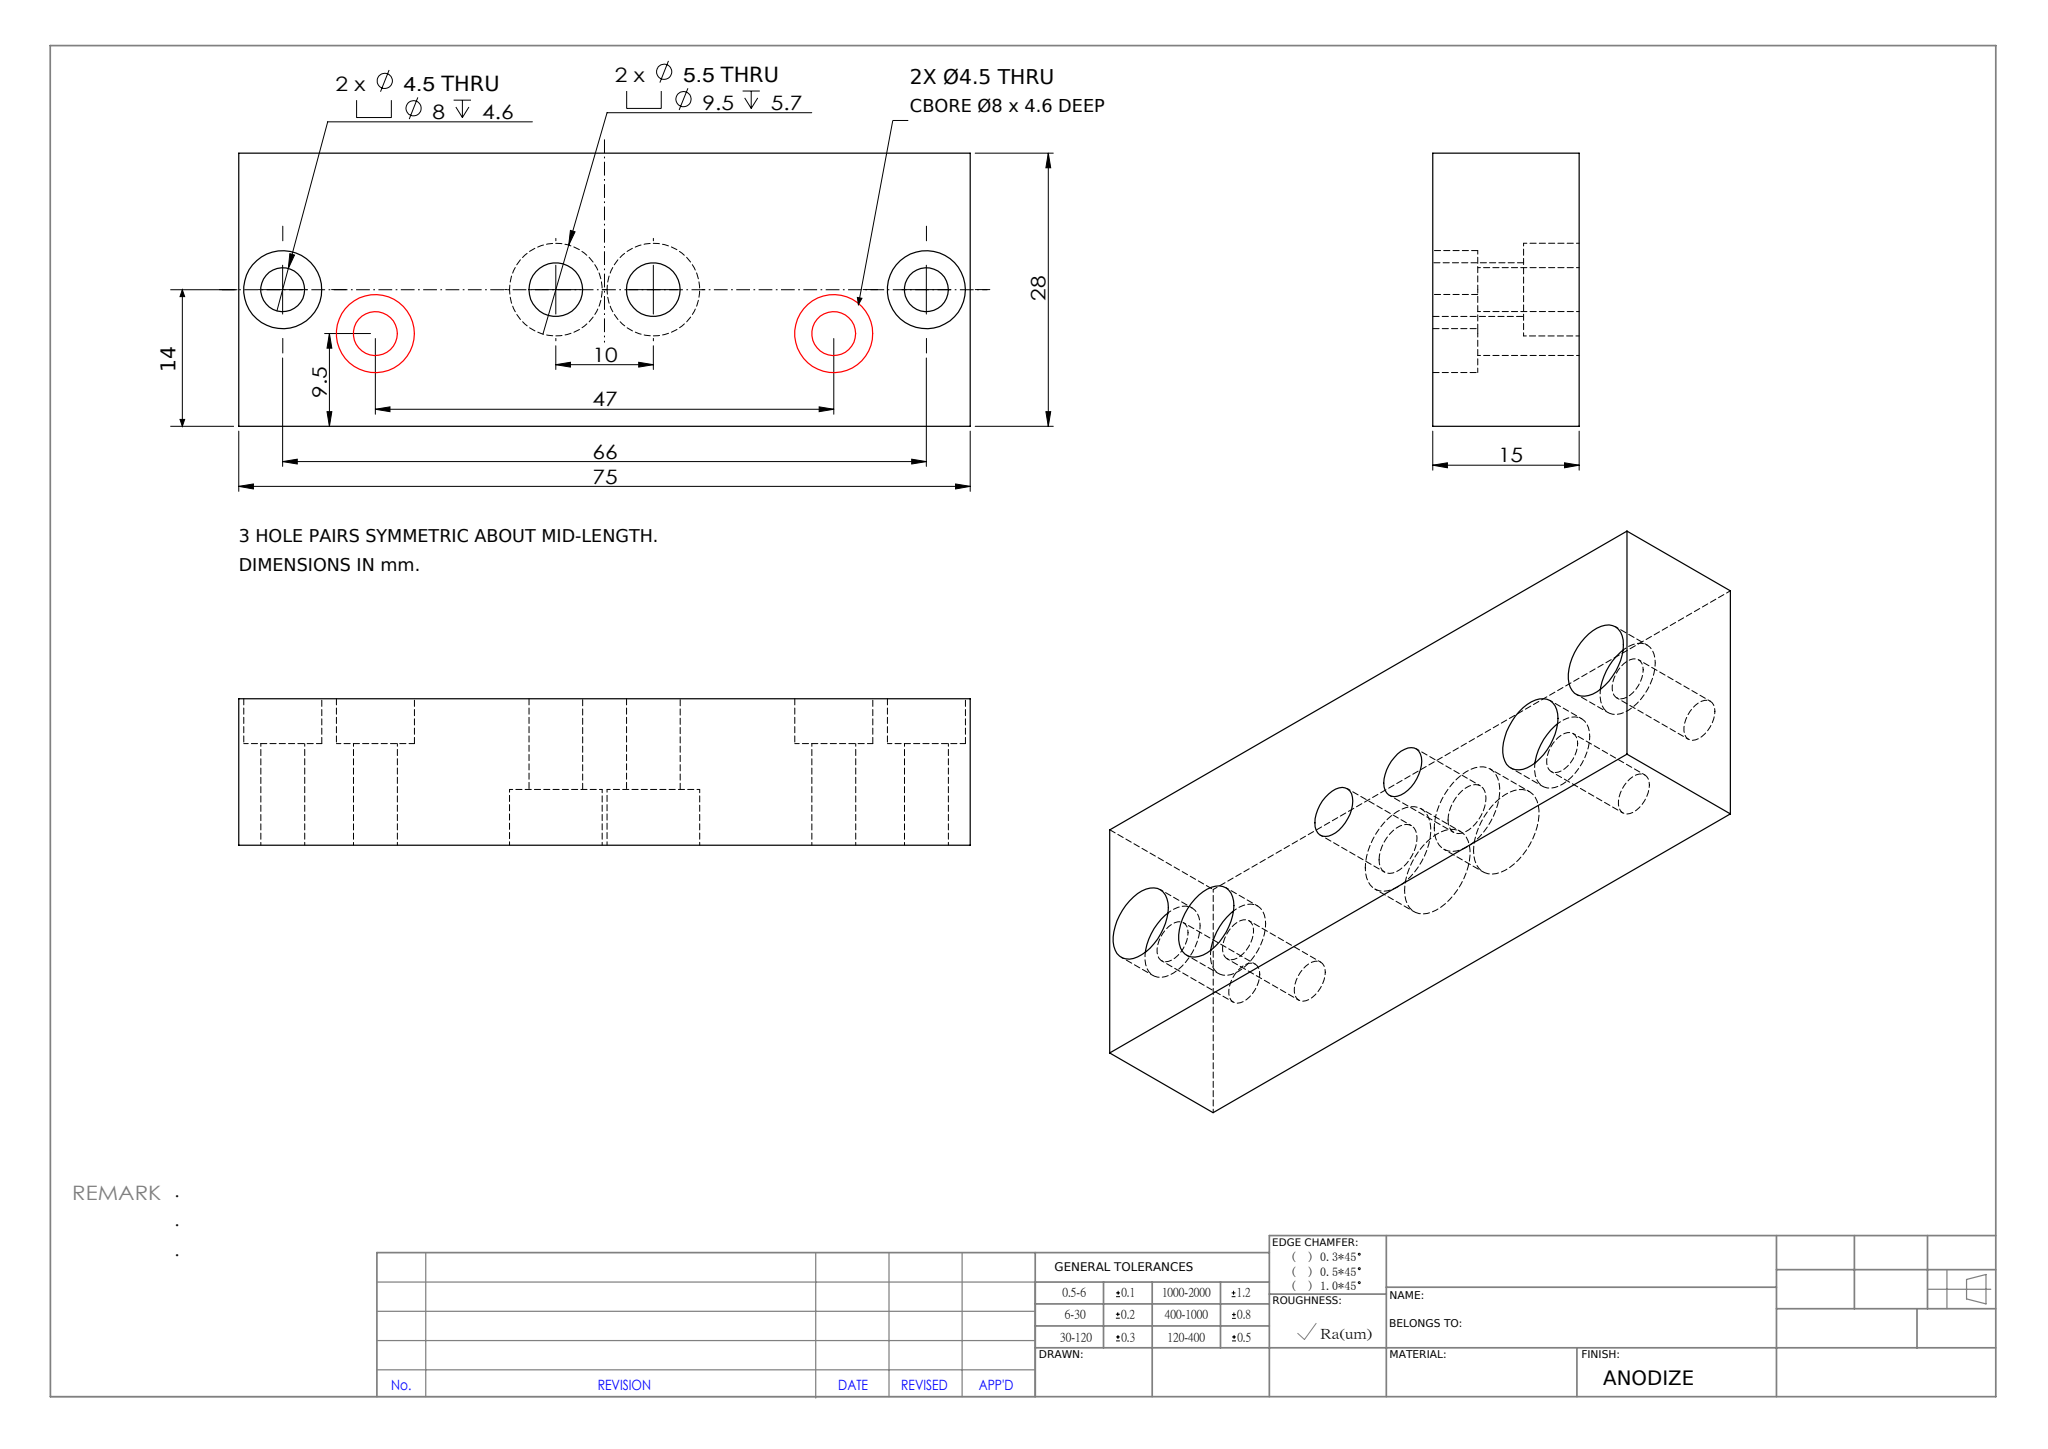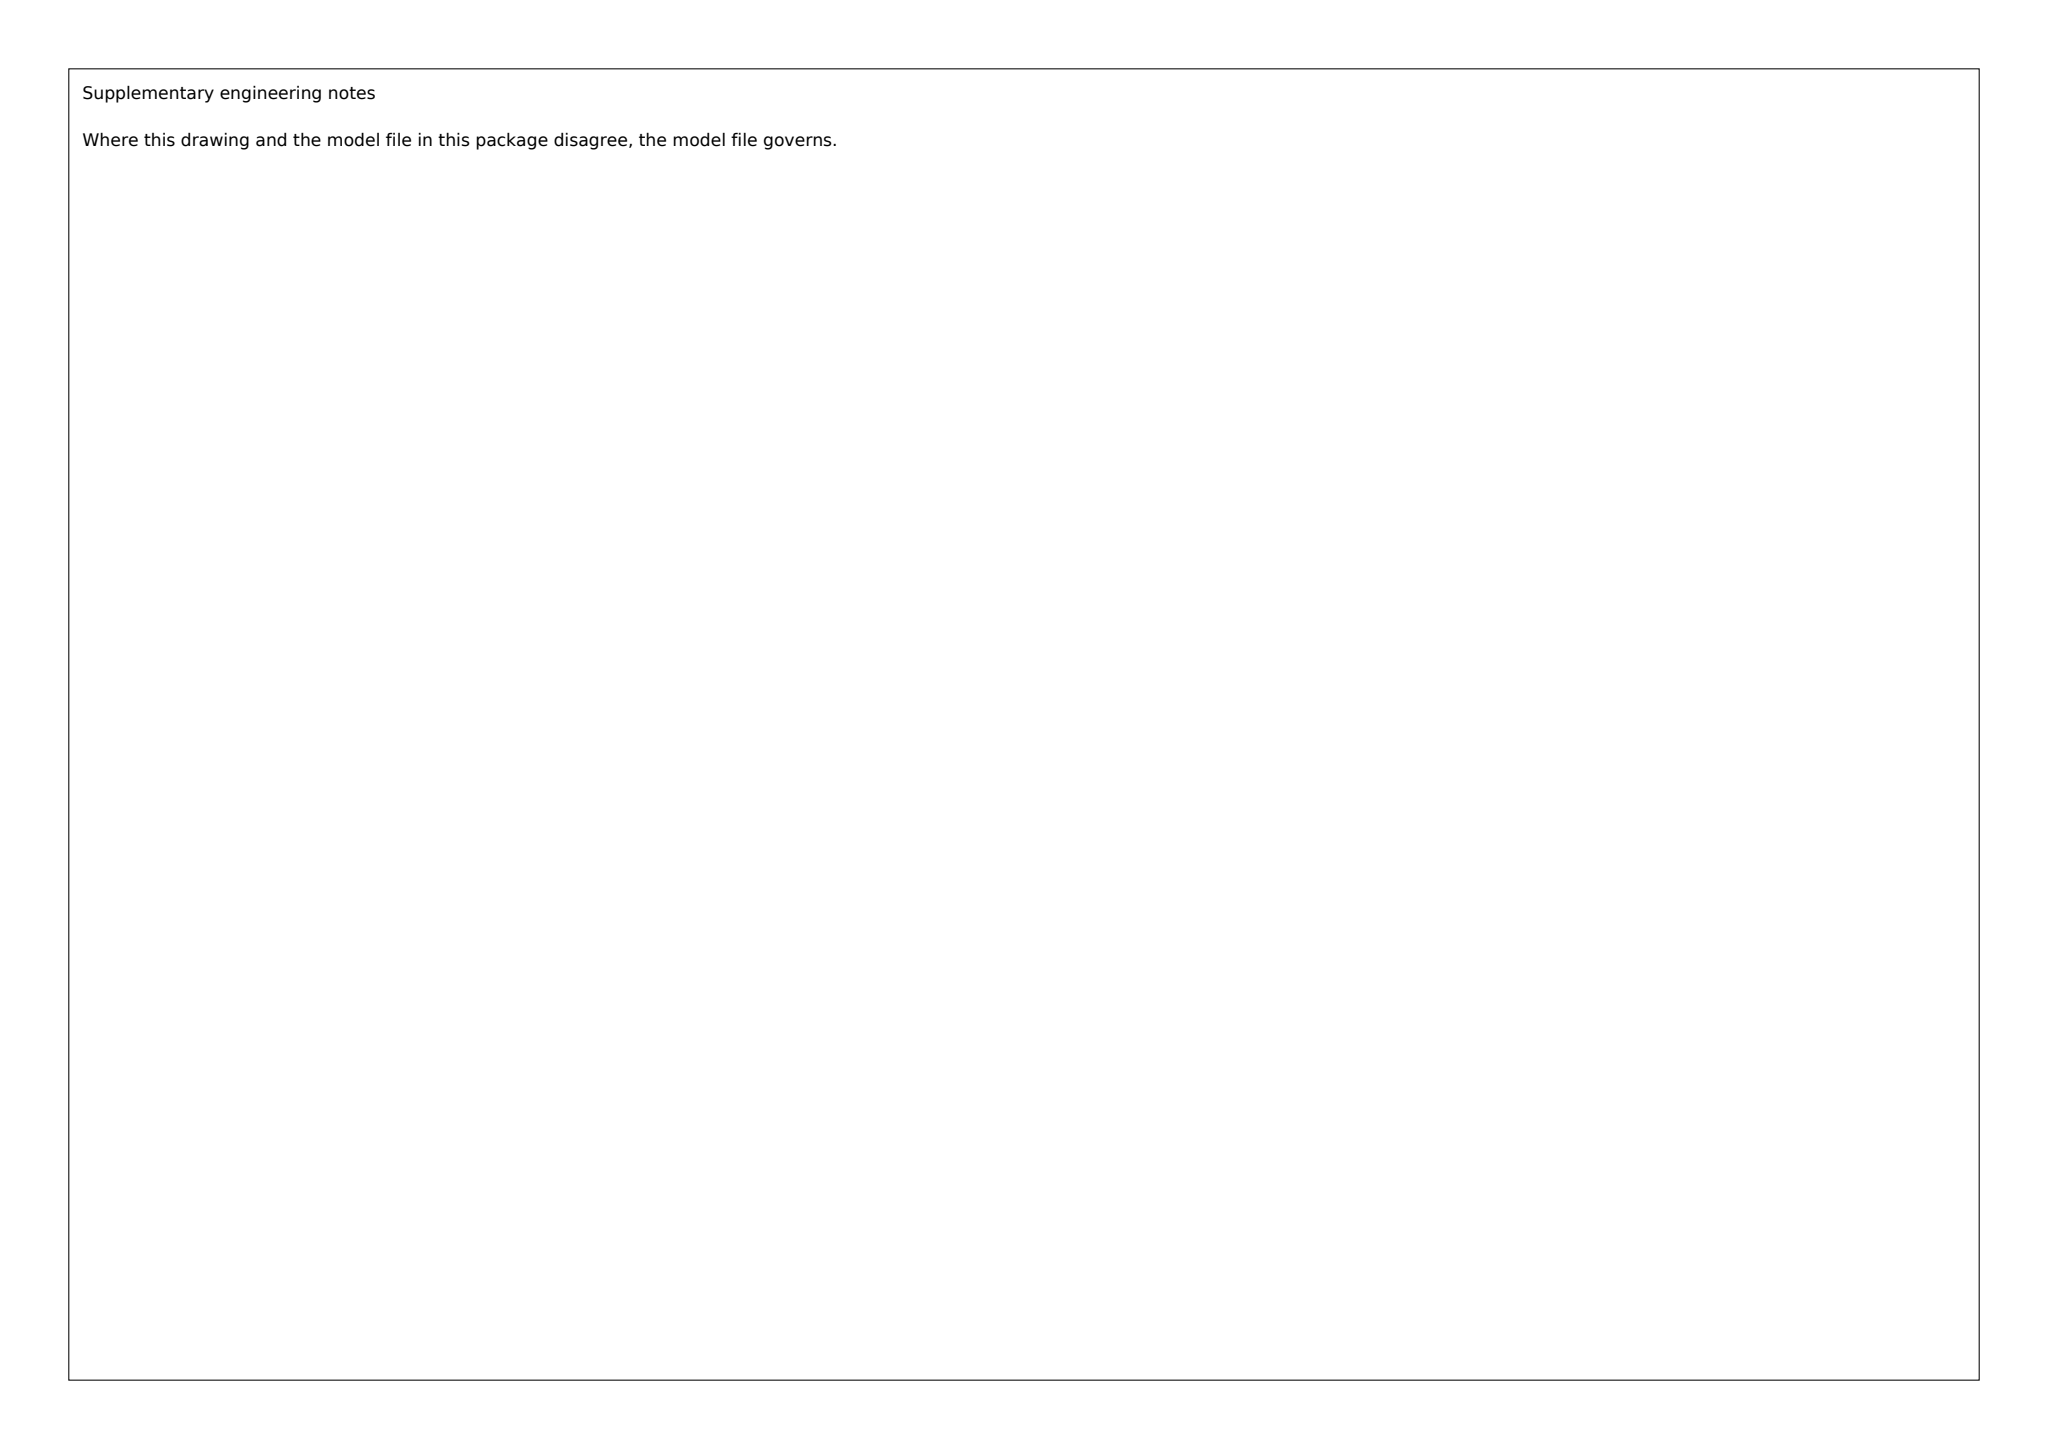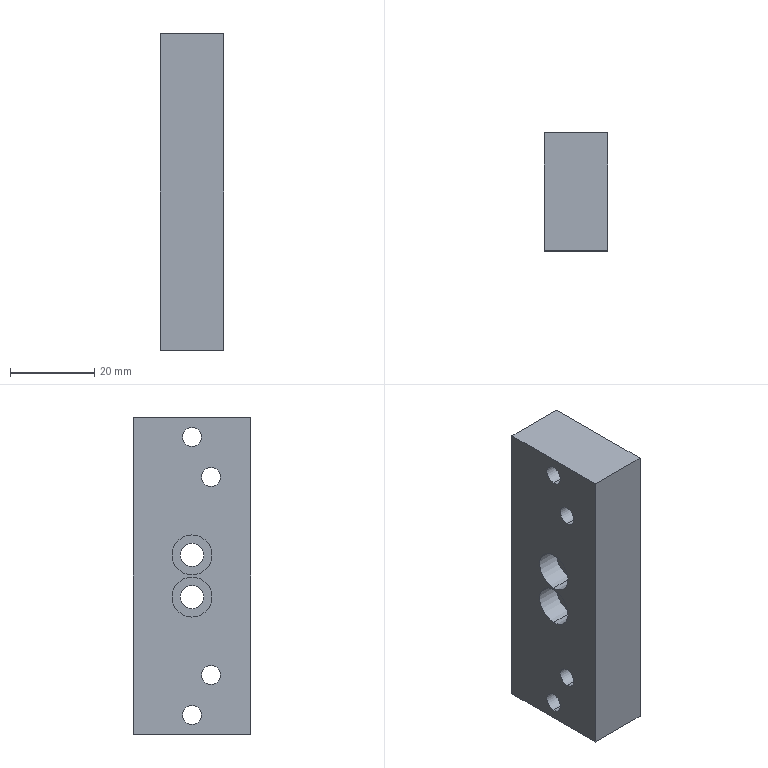Part | SolidWorks | mm | 1 solid | 36 faces | box 15 x 28 x 75 mm | volume 28664 mm3 | cylinder 24 | plane 12 | commonest cylinder face diameters 8 x8 4.5 x8 9.5 x4 5.5 x4
build123d program:
from build123d import *

# Parameters (mm, degrees)
SKETCH1_W                                         = 75
SKETCH1_H                                         = 28
BOSS_EXTRUDE1_DEPTH                               = 15
HOLE_SIZE_ACCORDING_TO_TYPE_2_FOR_HEX_D           = 4.5
HOLE_SIZE_ACCORDING_TO_TYPE_2_FOR_HEX_CBORE_D     = 8
HOLE_SIZE_ACCORDING_TO_TYPE_2_FOR_HEX_CBORE_DEPTH = 4.6
HOLE_SIZE_ACCORDING_TO_TYPE_2_FOR_2_D             = 5.5
HOLE_SIZE_ACCORDING_TO_TYPE_2_FOR_2_CBORE_D       = 9.5
HOLE_SIZE_ACCORDING_TO_TYPE_2_FOR_2_CBORE_DEPTH   = 5.7
HOLE_SIZE_ACCORDING_TO_TYPE_3_FOR_HEX_D           = 4.5
HOLE_SIZE_ACCORDING_TO_TYPE_3_FOR_HEX_CBORE_D     = 8
HOLE_SIZE_ACCORDING_TO_TYPE_3_FOR_HEX_CBORE_DEPTH = 4.6


with BuildPart() as part:
    # Sketch1 → Boss-Extrude1 (new body)
    with BuildSketch(Plane(origin=(0, 0, 0), x_dir=(0, 0, -1), z_dir=(1, 0, 0))):
        Rectangle(SKETCH1_W, SKETCH1_H)
    extrude(amount=BOSS_EXTRUDE1_DEPTH)

    # Hole Size _ according to_ Type 2 for Hex (through all)
    with Locations(Plane(origin=(15, 0, 0), x_dir=(0, 0, -1), z_dir=(1, 0, 0))):
        with Locations((-33, 0), (33, 0)):
            CounterBoreHole(HOLE_SIZE_ACCORDING_TO_TYPE_2_FOR_HEX_D / 2, HOLE_SIZE_ACCORDING_TO_TYPE_2_FOR_HEX_CBORE_D / 2, HOLE_SIZE_ACCORDING_TO_TYPE_2_FOR_HEX_CBORE_DEPTH)

    # Hole Size _ according to_ Type 2 for 2 (through all)
    with Locations(Plane.ZY):
        with Locations((-5, 0), (5, 0)):
            CounterBoreHole(HOLE_SIZE_ACCORDING_TO_TYPE_2_FOR_2_D / 2, HOLE_SIZE_ACCORDING_TO_TYPE_2_FOR_2_CBORE_D / 2, HOLE_SIZE_ACCORDING_TO_TYPE_2_FOR_2_CBORE_DEPTH)

    # Hole Size _ according to_ Type 3 for Hex (through all)
    with Locations(Plane(origin=(15, 0, 0), x_dir=(0, 0, -1), z_dir=(1, 0, 0))):
        with Locations((-23.5, -4.5), (23.5, -4.5)):
            CounterBoreHole(HOLE_SIZE_ACCORDING_TO_TYPE_3_FOR_HEX_D / 2, HOLE_SIZE_ACCORDING_TO_TYPE_3_FOR_HEX_CBORE_D / 2, HOLE_SIZE_ACCORDING_TO_TYPE_3_FOR_HEX_CBORE_DEPTH)


solid = part.part